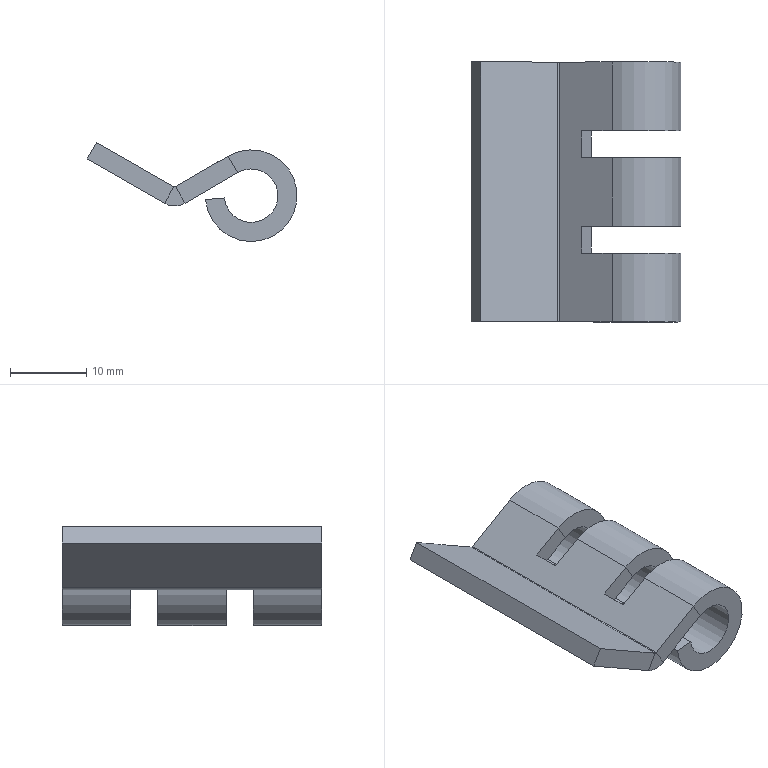Component | SolidWorks | FrontDoorFlangeWelding-2_CL201-1Hinge(ClawTypeAttachment)-1 | 1 solid | 34 faces | box 27.45 x 34 x 12.97 mm | volume 3368 mm3 | plane 26 | cylinder 8 | commonest cylinder face diameters 12 x3 7 x3 5.4 x1 0.4 x1
STEP:
#1=COLOUR_RGB('',0.7922,0.8196,0.9333);
#2=FILL_AREA_STYLE_COLOUR('',#1);
#3=FILL_AREA_STYLE('',(#2));
#4=SURFACE_STYLE_FILL_AREA(#3);
#5=SURFACE_SIDE_STYLE('',(#4));
#6=SURFACE_STYLE_USAGE(.BOTH.,#5);
#7=PRESENTATION_STYLE_ASSIGNMENT((#6));
#8=CARTESIAN_POINT('',(3.428,27.109,53.649));
#9=VERTEX_POINT('',#8);
#10=CARTESIAN_POINT('',(3.311,27.109,53.425));
#11=VERTEX_POINT('',#10);
#12=CARTESIAN_POINT('',(3.547,27.109,53.445));
#13=DIRECTION('',(0.,1.,0.));
#14=DIRECTION('',(-0.8677,0.,0.4971));
#15=AXIS2_PLACEMENT_3D('',#12,#13,#14);
#16=CIRCLE('',#15,0.2362);
#17=EDGE_CURVE('',#9,#11,#16,.T.);
#18=ORIENTED_EDGE('',*,*,#17,.T.);
#19=CARTESIAN_POINT('',(3.311,27.463,53.425));
#20=VERTEX_POINT('',#19);
#21=CARTESIAN_POINT('',(3.311,27.956,53.425));
#22=DIRECTION('',(-0.,-1.,-0.));
#23=VECTOR('',#22,39.37);
#24=LINE('',#21,#23);
#25=EDGE_CURVE('',#20,#11,#24,.T.);
#26=ORIENTED_EDGE('',*,*,#25,.F.);
#27=CARTESIAN_POINT('',(3.428,27.463,53.649));
#28=VERTEX_POINT('',#27);
#29=CARTESIAN_POINT('',(3.547,27.463,53.445));
#30=DIRECTION('',(-0.,-1.,-0.));
#31=DIRECTION('',(-0.8677,0.,0.4971));
#32=AXIS2_PLACEMENT_3D('',#29,#30,#31);
#33=CIRCLE('',#32,0.2362);
#34=EDGE_CURVE('',#20,#28,#33,.T.);
#35=ORIENTED_EDGE('',*,*,#34,.T.);
#36=CARTESIAN_POINT('',(3.428,27.956,53.649));
#37=DIRECTION('',(-0.,-1.,-0.));
#38=VECTOR('',#37,39.37);
#39=LINE('',#36,#38);
#40=EDGE_CURVE('',#28,#9,#39,.T.);
#41=ORIENTED_EDGE('',*,*,#40,.T.);
#42=EDGE_LOOP('',(#18,#26,#35,#41));
#43=FACE_OUTER_BOUND('',#42,.T.);
#44=CARTESIAN_POINT('',(3.547,27.956,53.445));
#45=DIRECTION('',(-0.,-1.,-0.));
#46=DIRECTION('',(-0.8677,0.,0.4971));
#47=AXIS2_PLACEMENT_3D('',#44,#45,#46);
#48=CYLINDRICAL_SURFACE('',#47,0.2362);
#49=ADVANCED_FACE('',(#43),#48,.T.);
#50=CARTESIAN_POINT('',(3.311,26.971,53.425));
#51=VERTEX_POINT('',#50);
#52=CARTESIAN_POINT('',(3.428,26.971,53.649));
#53=VERTEX_POINT('',#52);
#54=CARTESIAN_POINT('',(3.547,26.971,53.445));
#55=DIRECTION('',(-0.,-1.,-0.));
#56=DIRECTION('',(-0.8677,0.,0.4971));
#57=AXIS2_PLACEMENT_3D('',#54,#55,#56);
#58=CIRCLE('',#57,0.2362);
#59=EDGE_CURVE('',#51,#53,#58,.T.);
#60=ORIENTED_EDGE('',*,*,#59,.T.);
#61=CARTESIAN_POINT('',(3.428,26.617,53.649));
#62=VERTEX_POINT('',#61);
#63=CARTESIAN_POINT('',(3.428,27.956,53.649));
#64=DIRECTION('',(-0.,-1.,-0.));
#65=VECTOR('',#64,39.37);
#66=LINE('',#63,#65);
#67=EDGE_CURVE('',#53,#62,#66,.T.);
#68=ORIENTED_EDGE('',*,*,#67,.T.);
#69=CARTESIAN_POINT('',(3.311,26.617,53.425));
#70=VERTEX_POINT('',#69);
#71=CARTESIAN_POINT('',(3.547,26.617,53.445));
#72=DIRECTION('',(0.,1.,0.));
#73=DIRECTION('',(0.8677,0.,-0.4971));
#74=AXIS2_PLACEMENT_3D('',#71,#72,#73);
#75=CIRCLE('',#74,0.2362);
#76=EDGE_CURVE('',#62,#70,#75,.T.);
#77=ORIENTED_EDGE('',*,*,#76,.T.);
#78=CARTESIAN_POINT('',(3.311,27.956,53.425));
#79=DIRECTION('',(-0.,-1.,-0.));
#80=VECTOR('',#79,39.37);
#81=LINE('',#78,#80);
#82=EDGE_CURVE('',#51,#70,#81,.T.);
#83=ORIENTED_EDGE('',*,*,#82,.F.);
#84=EDGE_LOOP('',(#60,#68,#77,#83));
#85=FACE_OUTER_BOUND('',#84,.T.);
#86=CARTESIAN_POINT('',(3.547,27.956,53.445));
#87=DIRECTION('',(-0.,-1.,-0.));
#88=DIRECTION('',(-0.8677,0.,0.4971));
#89=AXIS2_PLACEMENT_3D('',#86,#87,#88);
#90=CYLINDRICAL_SURFACE('',#89,0.2362);
#91=ADVANCED_FACE('',(#85),#90,.T.);
#92=ORIENTED_EDGE('',*,*,#25,.T.);
#93=CARTESIAN_POINT('',(3.409,27.109,53.434));
#94=VERTEX_POINT('',#93);
#95=CARTESIAN_POINT('',(3.409,27.109,53.434));
#96=DIRECTION('',(-0.9965,0.,-0.08389));
#97=VECTOR('',#96,39.37);
#98=LINE('',#95,#97);
#99=EDGE_CURVE('',#94,#11,#98,.T.);
#100=ORIENTED_EDGE('',*,*,#99,.F.);
#101=CARTESIAN_POINT('',(3.409,27.463,53.434));
#102=VERTEX_POINT('',#101);
#103=CARTESIAN_POINT('',(3.409,27.956,53.434));
#104=DIRECTION('',(-0.,-1.,-0.));
#105=VECTOR('',#104,39.37);
#106=LINE('',#103,#105);
#107=EDGE_CURVE('',#102,#94,#106,.T.);
#108=ORIENTED_EDGE('',*,*,#107,.F.);
#109=CARTESIAN_POINT('',(3.409,27.463,53.434));
#110=DIRECTION('',(-0.9965,0.,-0.08389));
#111=VECTOR('',#110,39.37);
#112=LINE('',#109,#111);
#113=EDGE_CURVE('',#102,#20,#112,.T.);
#114=ORIENTED_EDGE('',*,*,#113,.T.);
#115=EDGE_LOOP('',(#92,#100,#108,#114));
#116=FACE_OUTER_BOUND('',#115,.T.);
#117=CARTESIAN_POINT('',(3.409,27.956,53.434));
#118=DIRECTION('',(-0.08389,-0.,0.9965));
#119=DIRECTION('',(0.9965,-0.,0.08389));
#120=AXIS2_PLACEMENT_3D('',#117,#118,#119);
#121=PLANE('',#120);
#122=ADVANCED_FACE('',(#116),#121,.T.);
#123=CARTESIAN_POINT('',(3.409,26.971,53.434));
#124=VERTEX_POINT('',#123);
#125=CARTESIAN_POINT('',(3.409,26.617,53.434));
#126=VERTEX_POINT('',#125);
#127=CARTESIAN_POINT('',(3.409,27.956,53.434));
#128=DIRECTION('',(-0.,-1.,-0.));
#129=VECTOR('',#128,39.37);
#130=LINE('',#127,#129);
#131=EDGE_CURVE('',#124,#126,#130,.T.);
#132=ORIENTED_EDGE('',*,*,#131,.F.);
#133=CARTESIAN_POINT('',(3.409,26.971,53.434));
#134=DIRECTION('',(-0.9965,0.,-0.08389));
#135=VECTOR('',#134,39.37);
#136=LINE('',#133,#135);
#137=EDGE_CURVE('',#124,#51,#136,.T.);
#138=ORIENTED_EDGE('',*,*,#137,.T.);
#139=ORIENTED_EDGE('',*,*,#82,.T.);
#140=CARTESIAN_POINT('',(3.409,26.617,53.434));
#141=DIRECTION('',(-0.9965,0.,-0.08389));
#142=VECTOR('',#141,39.37);
#143=LINE('',#140,#142);
#144=EDGE_CURVE('',#126,#70,#143,.T.);
#145=ORIENTED_EDGE('',*,*,#144,.F.);
#146=EDGE_LOOP('',(#132,#138,#139,#145));
#147=FACE_OUTER_BOUND('',#146,.T.);
#148=CARTESIAN_POINT('',(3.409,27.956,53.434));
#149=DIRECTION('',(-0.08389,-0.,0.9965));
#150=DIRECTION('',(0.9965,-0.,0.08389));
#151=AXIS2_PLACEMENT_3D('',#148,#149,#150);
#152=PLANE('',#151);
#153=ADVANCED_FACE('',(#147),#152,.T.);
#154=ORIENTED_EDGE('',*,*,#107,.T.);
#155=CARTESIAN_POINT('',(3.477,27.109,53.564));
#156=VERTEX_POINT('',#155);
#157=CARTESIAN_POINT('',(3.547,27.109,53.445));
#158=DIRECTION('',(0.,1.,0.));
#159=DIRECTION('',(0.8677,0.,-0.4971));
#160=AXIS2_PLACEMENT_3D('',#157,#158,#159);
#161=CIRCLE('',#160,0.1378);
#162=EDGE_CURVE('',#156,#94,#161,.T.);
#163=ORIENTED_EDGE('',*,*,#162,.F.);
#164=CARTESIAN_POINT('',(3.477,27.463,53.564));
#165=VERTEX_POINT('',#164);
#166=CARTESIAN_POINT('',(3.477,27.956,53.564));
#167=DIRECTION('',(-0.,-1.,-0.));
#168=VECTOR('',#167,39.37);
#169=LINE('',#166,#168);
#170=EDGE_CURVE('',#165,#156,#169,.T.);
#171=ORIENTED_EDGE('',*,*,#170,.F.);
#172=CARTESIAN_POINT('',(3.547,27.463,53.445));
#173=DIRECTION('',(-0.,-1.,-0.));
#174=DIRECTION('',(-0.8677,0.,0.4971));
#175=AXIS2_PLACEMENT_3D('',#172,#173,#174);
#176=CIRCLE('',#175,0.1378);
#177=EDGE_CURVE('',#102,#165,#176,.T.);
#178=ORIENTED_EDGE('',*,*,#177,.F.);
#179=EDGE_LOOP('',(#154,#163,#171,#178));
#180=FACE_OUTER_BOUND('',#179,.T.);
#181=CARTESIAN_POINT('',(3.547,27.956,53.445));
#182=DIRECTION('',(-0.,-1.,-0.));
#183=DIRECTION('',(-0.8677,0.,0.4971));
#184=AXIS2_PLACEMENT_3D('',#181,#182,#183);
#185=CYLINDRICAL_SURFACE('',#184,0.1378);
#186=ADVANCED_FACE('',(#180),#185,.F.);
#187=CARTESIAN_POINT('',(3.477,26.971,53.564));
#188=VERTEX_POINT('',#187);
#189=CARTESIAN_POINT('',(3.477,26.617,53.564));
#190=VERTEX_POINT('',#189);
#191=CARTESIAN_POINT('',(3.477,27.956,53.564));
#192=DIRECTION('',(-0.,-1.,-0.));
#193=VECTOR('',#192,39.37);
#194=LINE('',#191,#193);
#195=EDGE_CURVE('',#188,#190,#194,.T.);
#196=ORIENTED_EDGE('',*,*,#195,.F.);
#197=CARTESIAN_POINT('',(3.547,26.971,53.445));
#198=DIRECTION('',(0.,-1.,-0.));
#199=DIRECTION('',(-0.8677,0.,0.4971));
#200=AXIS2_PLACEMENT_3D('',#197,#198,#199);
#201=CIRCLE('',#200,0.1378);
#202=EDGE_CURVE('',#124,#188,#201,.T.);
#203=ORIENTED_EDGE('',*,*,#202,.F.);
#204=ORIENTED_EDGE('',*,*,#131,.T.);
#205=CARTESIAN_POINT('',(3.547,26.617,53.445));
#206=DIRECTION('',(0.,1.,0.));
#207=DIRECTION('',(0.8677,0.,-0.4971));
#208=AXIS2_PLACEMENT_3D('',#205,#206,#207);
#209=CIRCLE('',#208,0.1378);
#210=EDGE_CURVE('',#190,#126,#209,.T.);
#211=ORIENTED_EDGE('',*,*,#210,.F.);
#212=EDGE_LOOP('',(#196,#203,#204,#211));
#213=FACE_OUTER_BOUND('',#212,.T.);
#214=CARTESIAN_POINT('',(3.547,27.956,53.445));
#215=DIRECTION('',(-0.,-1.,-0.));
#216=DIRECTION('',(-0.8677,0.,0.4971));
#217=AXIS2_PLACEMENT_3D('',#214,#215,#216);
#218=CYLINDRICAL_SURFACE('',#217,0.1378);
#219=ADVANCED_FACE('',(#213),#218,.F.);
#220=ORIENTED_EDGE('',*,*,#170,.T.);
#221=CARTESIAN_POINT('',(3.32,27.109,53.473));
#222=VERTEX_POINT('',#221);
#223=CARTESIAN_POINT('',(3.153,27.109,53.376));
#224=DIRECTION('',(0.8644,-0.,0.5029));
#225=VECTOR('',#224,39.37);
#226=LINE('',#223,#225);
#227=EDGE_CURVE('',#222,#156,#226,.T.);
#228=ORIENTED_EDGE('',*,*,#227,.F.);
#229=CARTESIAN_POINT('',(3.32,26.971,53.473));
#230=VERTEX_POINT('',#229);
#231=CARTESIAN_POINT('',(3.32,27.956,53.473));
#232=DIRECTION('',(0.,1.,0.));
#233=VECTOR('',#232,39.37);
#234=LINE('',#231,#233);
#235=EDGE_CURVE('',#230,#222,#234,.T.);
#236=ORIENTED_EDGE('',*,*,#235,.F.);
#237=CARTESIAN_POINT('',(3.153,26.971,53.376));
#238=DIRECTION('',(-0.8644,0.,-0.5029));
#239=VECTOR('',#238,39.37);
#240=LINE('',#237,#239);
#241=EDGE_CURVE('',#188,#230,#240,.T.);
#242=ORIENTED_EDGE('',*,*,#241,.F.);
#243=ORIENTED_EDGE('',*,*,#195,.T.);
#244=CARTESIAN_POINT('',(3.206,26.617,53.406));
#245=VERTEX_POINT('',#244);
#246=CARTESIAN_POINT('',(3.153,26.617,53.376));
#247=DIRECTION('',(0.8644,-0.,0.5029));
#248=VECTOR('',#247,39.37);
#249=LINE('',#246,#248);
#250=EDGE_CURVE('',#245,#190,#249,.T.);
#251=ORIENTED_EDGE('',*,*,#250,.F.);
#252=CARTESIAN_POINT('',(3.206,27.956,53.406));
#253=VERTEX_POINT('',#252);
#254=CARTESIAN_POINT('',(3.206,27.956,53.406));
#255=DIRECTION('',(-0.,-1.,-0.));
#256=VECTOR('',#255,39.37);
#257=LINE('',#254,#256);
#258=EDGE_CURVE('',#253,#245,#257,.T.);
#259=ORIENTED_EDGE('',*,*,#258,.F.);
#260=CARTESIAN_POINT('',(3.477,27.956,53.564));
#261=VERTEX_POINT('',#260);
#262=CARTESIAN_POINT('',(3.153,27.956,53.376));
#263=DIRECTION('',(0.8644,-0.,0.5029));
#264=VECTOR('',#263,39.37);
#265=LINE('',#262,#264);
#266=EDGE_CURVE('',#253,#261,#265,.T.);
#267=ORIENTED_EDGE('',*,*,#266,.T.);
#268=CARTESIAN_POINT('',(3.477,27.601,53.564));
#269=VERTEX_POINT('',#268);
#270=CARTESIAN_POINT('',(3.477,27.956,53.564));
#271=DIRECTION('',(-0.,-1.,-0.));
#272=VECTOR('',#271,39.37);
#273=LINE('',#270,#272);
#274=EDGE_CURVE('',#261,#269,#273,.T.);
#275=ORIENTED_EDGE('',*,*,#274,.T.);
#276=CARTESIAN_POINT('',(3.32,27.601,53.473));
#277=VERTEX_POINT('',#276);
#278=CARTESIAN_POINT('',(3.153,27.601,53.376));
#279=DIRECTION('',(0.8644,-0.,0.5029));
#280=VECTOR('',#279,39.37);
#281=LINE('',#278,#280);
#282=EDGE_CURVE('',#277,#269,#281,.T.);
#283=ORIENTED_EDGE('',*,*,#282,.F.);
#284=CARTESIAN_POINT('',(3.32,27.463,53.473));
#285=VERTEX_POINT('',#284);
#286=CARTESIAN_POINT('',(3.32,27.956,53.473));
#287=DIRECTION('',(-0.,1.,0.));
#288=VECTOR('',#287,39.37);
#289=LINE('',#286,#288);
#290=EDGE_CURVE('',#285,#277,#289,.T.);
#291=ORIENTED_EDGE('',*,*,#290,.F.);
#292=CARTESIAN_POINT('',(3.153,27.463,53.376));
#293=DIRECTION('',(-0.8644,0.,-0.5029));
#294=VECTOR('',#293,39.37);
#295=LINE('',#292,#294);
#296=EDGE_CURVE('',#165,#285,#295,.T.);
#297=ORIENTED_EDGE('',*,*,#296,.F.);
#298=EDGE_LOOP('',(#220,#228,#236,#242,#243,#251,#259,#267,#275,#283,#291,#297));
#299=FACE_OUTER_BOUND('',#298,.T.);
#300=CARTESIAN_POINT('',(3.153,27.956,53.376));
#301=DIRECTION('',(0.5029,0.,-0.8644));
#302=DIRECTION('',(-0.8644,0.,-0.5029));
#303=AXIS2_PLACEMENT_3D('',#300,#301,#302);
#304=PLANE('',#303);
#305=ADVANCED_FACE('',(#299),#304,.T.);
#306=CARTESIAN_POINT('',(3.271,27.109,53.558));
#307=VERTEX_POINT('',#306);
#308=CARTESIAN_POINT('',(3.104,27.109,53.461));
#309=DIRECTION('',(0.8644,-0.,0.5029));
#310=VECTOR('',#309,39.37);
#311=LINE('',#308,#310);
#312=EDGE_CURVE('',#307,#9,#311,.T.);
#313=ORIENTED_EDGE('',*,*,#312,.T.);
#314=ORIENTED_EDGE('',*,*,#40,.F.);
#315=CARTESIAN_POINT('',(3.271,27.463,53.558));
#316=VERTEX_POINT('',#315);
#317=CARTESIAN_POINT('',(3.104,27.463,53.461));
#318=DIRECTION('',(-0.8644,0.,-0.5029));
#319=VECTOR('',#318,39.37);
#320=LINE('',#317,#319);
#321=EDGE_CURVE('',#28,#316,#320,.T.);
#322=ORIENTED_EDGE('',*,*,#321,.T.);
#323=CARTESIAN_POINT('',(3.271,27.601,53.558));
#324=VERTEX_POINT('',#323);
#325=CARTESIAN_POINT('',(3.271,27.956,53.558));
#326=DIRECTION('',(0.,1.,0.));
#327=VECTOR('',#326,39.37);
#328=LINE('',#325,#327);
#329=EDGE_CURVE('',#316,#324,#328,.T.);
#330=ORIENTED_EDGE('',*,*,#329,.T.);
#331=CARTESIAN_POINT('',(3.428,27.601,53.649));
#332=VERTEX_POINT('',#331);
#333=CARTESIAN_POINT('',(3.104,27.601,53.461));
#334=DIRECTION('',(0.8644,-0.,0.5029));
#335=VECTOR('',#334,39.37);
#336=LINE('',#333,#335);
#337=EDGE_CURVE('',#324,#332,#336,.T.);
#338=ORIENTED_EDGE('',*,*,#337,.T.);
#339=CARTESIAN_POINT('',(3.428,27.956,53.649));
#340=VERTEX_POINT('',#339);
#341=CARTESIAN_POINT('',(3.428,27.956,53.649));
#342=DIRECTION('',(-0.,-1.,-0.));
#343=VECTOR('',#342,39.37);
#344=LINE('',#341,#343);
#345=EDGE_CURVE('',#340,#332,#344,.T.);
#346=ORIENTED_EDGE('',*,*,#345,.F.);
#347=CARTESIAN_POINT('',(3.157,27.956,53.492));
#348=VERTEX_POINT('',#347);
#349=CARTESIAN_POINT('',(3.104,27.956,53.461));
#350=DIRECTION('',(0.8644,-0.,0.5029));
#351=VECTOR('',#350,39.37);
#352=LINE('',#349,#351);
#353=EDGE_CURVE('',#348,#340,#352,.T.);
#354=ORIENTED_EDGE('',*,*,#353,.F.);
#355=CARTESIAN_POINT('',(3.157,26.617,53.492));
#356=VERTEX_POINT('',#355);
#357=CARTESIAN_POINT('',(3.157,27.956,53.492));
#358=DIRECTION('',(-0.,-1.,-0.));
#359=VECTOR('',#358,39.37);
#360=LINE('',#357,#359);
#361=EDGE_CURVE('',#348,#356,#360,.T.);
#362=ORIENTED_EDGE('',*,*,#361,.T.);
#363=CARTESIAN_POINT('',(3.104,26.617,53.461));
#364=DIRECTION('',(0.8644,-0.,0.5029));
#365=VECTOR('',#364,39.37);
#366=LINE('',#363,#365);
#367=EDGE_CURVE('',#356,#62,#366,.T.);
#368=ORIENTED_EDGE('',*,*,#367,.T.);
#369=ORIENTED_EDGE('',*,*,#67,.F.);
#370=CARTESIAN_POINT('',(3.271,26.971,53.558));
#371=VERTEX_POINT('',#370);
#372=CARTESIAN_POINT('',(3.104,26.971,53.461));
#373=DIRECTION('',(-0.8644,0.,-0.5029));
#374=VECTOR('',#373,39.37);
#375=LINE('',#372,#374);
#376=EDGE_CURVE('',#53,#371,#375,.T.);
#377=ORIENTED_EDGE('',*,*,#376,.T.);
#378=CARTESIAN_POINT('',(3.271,27.956,53.558));
#379=DIRECTION('',(0.,1.,0.));
#380=VECTOR('',#379,39.37);
#381=LINE('',#378,#380);
#382=EDGE_CURVE('',#371,#307,#381,.T.);
#383=ORIENTED_EDGE('',*,*,#382,.T.);
#384=EDGE_LOOP('',(#313,#314,#322,#330,#338,#346,#354,#362,#368,#369,#377,#383));
#385=FACE_OUTER_BOUND('',#384,.T.);
#386=CARTESIAN_POINT('',(3.104,27.956,53.461));
#387=DIRECTION('',(0.5029,0.,-0.8644));
#388=DIRECTION('',(-0.8644,0.,-0.5029));
#389=AXIS2_PLACEMENT_3D('',#386,#387,#388);
#390=PLANE('',#389);
#391=ADVANCED_FACE('',(#385),#390,.F.);
#392=CARTESIAN_POINT('',(3.311,27.601,53.425));
#393=VERTEX_POINT('',#392);
#394=CARTESIAN_POINT('',(3.547,27.601,53.445));
#395=DIRECTION('',(0.,1.,0.));
#396=DIRECTION('',(-0.8677,0.,0.4971));
#397=AXIS2_PLACEMENT_3D('',#394,#395,#396);
#398=CIRCLE('',#397,0.2362);
#399=EDGE_CURVE('',#332,#393,#398,.T.);
#400=ORIENTED_EDGE('',*,*,#399,.T.);
#401=CARTESIAN_POINT('',(3.311,27.956,53.425));
#402=VERTEX_POINT('',#401);
#403=CARTESIAN_POINT('',(3.311,27.956,53.425));
#404=DIRECTION('',(-0.,-1.,-0.));
#405=VECTOR('',#404,39.37);
#406=LINE('',#403,#405);
#407=EDGE_CURVE('',#402,#393,#406,.T.);
#408=ORIENTED_EDGE('',*,*,#407,.F.);
#409=CARTESIAN_POINT('',(3.547,27.956,53.445));
#410=DIRECTION('',(0.,1.,0.));
#411=DIRECTION('',(0.8677,0.,-0.4971));
#412=AXIS2_PLACEMENT_3D('',#409,#410,#411);
#413=CIRCLE('',#412,0.2362);
#414=EDGE_CURVE('',#340,#402,#413,.T.);
#415=ORIENTED_EDGE('',*,*,#414,.F.);
#416=ORIENTED_EDGE('',*,*,#345,.T.);
#417=EDGE_LOOP('',(#400,#408,#415,#416));
#418=FACE_OUTER_BOUND('',#417,.T.);
#419=CARTESIAN_POINT('',(3.547,27.956,53.445));
#420=DIRECTION('',(-0.,-1.,-0.));
#421=DIRECTION('',(-0.8677,0.,0.4971));
#422=AXIS2_PLACEMENT_3D('',#419,#420,#421);
#423=CYLINDRICAL_SURFACE('',#422,0.2362);
#424=ADVANCED_FACE('',(#418),#423,.T.);
#425=ORIENTED_EDGE('',*,*,#407,.T.);
#426=CARTESIAN_POINT('',(3.409,27.601,53.434));
#427=VERTEX_POINT('',#426);
#428=CARTESIAN_POINT('',(3.409,27.601,53.434));
#429=DIRECTION('',(-0.9965,0.,-0.08389));
#430=VECTOR('',#429,39.37);
#431=LINE('',#428,#430);
#432=EDGE_CURVE('',#427,#393,#431,.T.);
#433=ORIENTED_EDGE('',*,*,#432,.F.);
#434=CARTESIAN_POINT('',(3.409,27.956,53.434));
#435=VERTEX_POINT('',#434);
#436=CARTESIAN_POINT('',(3.409,27.956,53.434));
#437=DIRECTION('',(-0.,-1.,-0.));
#438=VECTOR('',#437,39.37);
#439=LINE('',#436,#438);
#440=EDGE_CURVE('',#435,#427,#439,.T.);
#441=ORIENTED_EDGE('',*,*,#440,.F.);
#442=CARTESIAN_POINT('',(3.409,27.956,53.434));
#443=DIRECTION('',(-0.9965,0.,-0.08389));
#444=VECTOR('',#443,39.37);
#445=LINE('',#442,#444);
#446=EDGE_CURVE('',#435,#402,#445,.T.);
#447=ORIENTED_EDGE('',*,*,#446,.T.);
#448=EDGE_LOOP('',(#425,#433,#441,#447));
#449=FACE_OUTER_BOUND('',#448,.T.);
#450=CARTESIAN_POINT('',(3.409,27.956,53.434));
#451=DIRECTION('',(-0.08389,-0.,0.9965));
#452=DIRECTION('',(0.9965,-0.,0.08389));
#453=AXIS2_PLACEMENT_3D('',#450,#451,#452);
#454=PLANE('',#453);
#455=ADVANCED_FACE('',(#449),#454,.T.);
#456=ORIENTED_EDGE('',*,*,#440,.T.);
#457=CARTESIAN_POINT('',(3.547,27.601,53.445));
#458=DIRECTION('',(0.,1.,0.));
#459=DIRECTION('',(0.8677,0.,-0.4971));
#460=AXIS2_PLACEMENT_3D('',#457,#458,#459);
#461=CIRCLE('',#460,0.1378);
#462=EDGE_CURVE('',#269,#427,#461,.T.);
#463=ORIENTED_EDGE('',*,*,#462,.F.);
#464=ORIENTED_EDGE('',*,*,#274,.F.);
#465=CARTESIAN_POINT('',(3.547,27.956,53.445));
#466=DIRECTION('',(0.,1.,0.));
#467=DIRECTION('',(0.8677,0.,-0.4971));
#468=AXIS2_PLACEMENT_3D('',#465,#466,#467);
#469=CIRCLE('',#468,0.1378);
#470=EDGE_CURVE('',#261,#435,#469,.T.);
#471=ORIENTED_EDGE('',*,*,#470,.T.);
#472=EDGE_LOOP('',(#456,#463,#464,#471));
#473=FACE_OUTER_BOUND('',#472,.T.);
#474=CARTESIAN_POINT('',(3.547,27.956,53.445));
#475=DIRECTION('',(-0.,-1.,-0.));
#476=DIRECTION('',(-0.8677,0.,0.4971));
#477=AXIS2_PLACEMENT_3D('',#474,#475,#476);
#478=CYLINDRICAL_SURFACE('',#477,0.1378);
#479=ADVANCED_FACE('',(#473),#478,.F.);
#480=CARTESIAN_POINT('',(3.428,27.956,53.649));
#481=DIRECTION('',(0.5029,0.,-0.8644));
#482=VECTOR('',#481,39.37);
#483=LINE('',#480,#482);
#484=EDGE_CURVE('',#340,#261,#483,.T.);
#485=ORIENTED_EDGE('',*,*,#484,.F.);
#486=ORIENTED_EDGE('',*,*,#414,.T.);
#487=ORIENTED_EDGE('',*,*,#446,.F.);
#488=ORIENTED_EDGE('',*,*,#470,.F.);
#489=EDGE_LOOP('',(#485,#486,#487,#488));
#490=FACE_OUTER_BOUND('',#489,.T.);
#491=CARTESIAN_POINT('',(3.428,27.956,53.649));
#492=DIRECTION('',(0.,1.,0.));
#493=DIRECTION('',(0.8677,0.,-0.4971));
#494=AXIS2_PLACEMENT_3D('',#491,#492,#493);
#495=PLANE('',#494);
#496=ADVANCED_FACE('',(#490),#495,.T.);
#497=CARTESIAN_POINT('',(3.477,26.617,53.564));
#498=DIRECTION('',(-0.5029,-0.,0.8644));
#499=VECTOR('',#498,39.37);
#500=LINE('',#497,#499);
#501=EDGE_CURVE('',#190,#62,#500,.T.);
#502=ORIENTED_EDGE('',*,*,#501,.F.);
#503=ORIENTED_EDGE('',*,*,#210,.T.);
#504=ORIENTED_EDGE('',*,*,#144,.T.);
#505=ORIENTED_EDGE('',*,*,#76,.F.);
#506=EDGE_LOOP('',(#502,#503,#504,#505));
#507=FACE_OUTER_BOUND('',#506,.T.);
#508=CARTESIAN_POINT('',(3.477,26.617,53.564));
#509=DIRECTION('',(-0.,-1.,-0.));
#510=DIRECTION('',(-0.8677,-0.,0.4971));
#511=AXIS2_PLACEMENT_3D('',#508,#509,#510);
#512=PLANE('',#511);
#513=ADVANCED_FACE('',(#507),#512,.T.);
#514=CARTESIAN_POINT('',(3.206,27.956,53.406));
#515=DIRECTION('',(-0.5029,-0.,0.8644));
#516=VECTOR('',#515,39.37);
#517=LINE('',#514,#516);
#518=EDGE_CURVE('',#253,#348,#517,.T.);
#519=ORIENTED_EDGE('',*,*,#518,.F.);
#520=CARTESIAN_POINT('',(3.1,27.956,53.406));
#521=VERTEX_POINT('',#520);
#522=CARTESIAN_POINT('',(3.153,27.956,53.498));
#523=DIRECTION('',(-0.,-1.,-0.));
#524=DIRECTION('',(0.8677,0.,-0.4971));
#525=AXIS2_PLACEMENT_3D('',#522,#523,#524);
#526=CIRCLE('',#525,0.1063);
#527=EDGE_CURVE('',#521,#253,#526,.T.);
#528=ORIENTED_EDGE('',*,*,#527,.F.);
#529=CARTESIAN_POINT('',(3.149,27.956,53.492));
#530=VERTEX_POINT('',#529);
#531=CARTESIAN_POINT('',(3.149,27.956,53.492));
#532=DIRECTION('',(-0.4971,0.,-0.8677));
#533=VECTOR('',#532,39.37);
#534=LINE('',#531,#533);
#535=EDGE_CURVE('',#530,#521,#534,.T.);
#536=ORIENTED_EDGE('',*,*,#535,.F.);
#537=CARTESIAN_POINT('',(3.153,27.956,53.498));
#538=DIRECTION('',(-0.,-1.,-0.));
#539=DIRECTION('',(0.8677,0.,-0.4971));
#540=AXIS2_PLACEMENT_3D('',#537,#538,#539);
#541=CIRCLE('',#540,0.007874);
#542=EDGE_CURVE('',#530,#348,#541,.T.);
#543=ORIENTED_EDGE('',*,*,#542,.T.);
#544=EDGE_LOOP('',(#519,#528,#536,#543));
#545=FACE_OUTER_BOUND('',#544,.T.);
#546=CARTESIAN_POINT('',(3.206,27.956,53.406));
#547=DIRECTION('',(0.,1.,0.));
#548=DIRECTION('',(0.8677,0.,-0.4971));
#549=AXIS2_PLACEMENT_3D('',#546,#547,#548);
#550=PLANE('',#549);
#551=ADVANCED_FACE('',(#545),#550,.T.);
#552=ORIENTED_EDGE('',*,*,#266,.F.);
#553=ORIENTED_EDGE('',*,*,#518,.T.);
#554=ORIENTED_EDGE('',*,*,#353,.T.);
#555=ORIENTED_EDGE('',*,*,#484,.T.);
#556=EDGE_LOOP('',(#552,#553,#554,#555));
#557=FACE_OUTER_BOUND('',#556,.T.);
#558=CARTESIAN_POINT('',(3.149,27.956,53.492));
#559=DIRECTION('',(0.,1.,0.));
#560=DIRECTION('',(0.8677,0.,-0.4971));
#561=AXIS2_PLACEMENT_3D('',#558,#559,#560);
#562=PLANE('',#561);
#563=ADVANCED_FACE('',(#557),#562,.T.);
#564=CARTESIAN_POINT('',(3.1,26.617,53.406));
#565=VERTEX_POINT('',#564);
#566=CARTESIAN_POINT('',(3.149,26.617,53.492));
#567=VERTEX_POINT('',#566);
#568=CARTESIAN_POINT('',(3.1,26.617,53.406));
#569=DIRECTION('',(0.4971,-0.,0.8677));
#570=VECTOR('',#569,39.37);
#571=LINE('',#568,#570);
#572=EDGE_CURVE('',#565,#567,#571,.T.);
#573=ORIENTED_EDGE('',*,*,#572,.F.);
#574=CARTESIAN_POINT('',(3.153,26.617,53.498));
#575=DIRECTION('',(-0.,-1.,-0.));
#576=DIRECTION('',(0.8677,0.,-0.4971));
#577=AXIS2_PLACEMENT_3D('',#574,#575,#576);
#578=CIRCLE('',#577,0.1063);
#579=EDGE_CURVE('',#565,#245,#578,.T.);
#580=ORIENTED_EDGE('',*,*,#579,.T.);
#581=CARTESIAN_POINT('',(3.157,26.617,53.492));
#582=DIRECTION('',(0.5029,0.,-0.8644));
#583=VECTOR('',#582,39.37);
#584=LINE('',#581,#583);
#585=EDGE_CURVE('',#356,#245,#584,.T.);
#586=ORIENTED_EDGE('',*,*,#585,.F.);
#587=CARTESIAN_POINT('',(3.153,26.617,53.498));
#588=DIRECTION('',(-0.,-1.,-0.));
#589=DIRECTION('',(0.8677,0.,-0.4971));
#590=AXIS2_PLACEMENT_3D('',#587,#588,#589);
#591=CIRCLE('',#590,0.007874);
#592=EDGE_CURVE('',#567,#356,#591,.T.);
#593=ORIENTED_EDGE('',*,*,#592,.F.);
#594=EDGE_LOOP('',(#573,#580,#586,#593));
#595=FACE_OUTER_BOUND('',#594,.T.);
#596=CARTESIAN_POINT('',(3.1,26.617,53.406));
#597=DIRECTION('',(-0.,-1.,-0.));
#598=DIRECTION('',(-0.8677,-0.,0.4971));
#599=AXIS2_PLACEMENT_3D('',#596,#597,#598);
#600=PLANE('',#599);
#601=ADVANCED_FACE('',(#595),#600,.T.);
#602=CARTESIAN_POINT('',(2.702,26.617,53.634));
#603=VERTEX_POINT('',#602);
#604=CARTESIAN_POINT('',(2.702,26.617,53.634));
#605=DIRECTION('',(0.8677,0.,-0.4971));
#606=VECTOR('',#605,39.37);
#607=LINE('',#604,#606);
#608=EDGE_CURVE('',#603,#565,#607,.T.);
#609=ORIENTED_EDGE('',*,*,#608,.T.);
#610=ORIENTED_EDGE('',*,*,#572,.T.);
#611=CARTESIAN_POINT('',(2.751,26.617,53.719));
#612=VERTEX_POINT('',#611);
#613=CARTESIAN_POINT('',(2.751,26.617,53.719));
#614=DIRECTION('',(0.8677,0.,-0.4971));
#615=VECTOR('',#614,39.37);
#616=LINE('',#613,#615);
#617=EDGE_CURVE('',#612,#567,#616,.T.);
#618=ORIENTED_EDGE('',*,*,#617,.F.);
#619=CARTESIAN_POINT('',(2.751,26.617,53.719));
#620=DIRECTION('',(-0.4971,0.,-0.8677));
#621=VECTOR('',#620,39.37);
#622=LINE('',#619,#621);
#623=EDGE_CURVE('',#612,#603,#622,.T.);
#624=ORIENTED_EDGE('',*,*,#623,.T.);
#625=EDGE_LOOP('',(#609,#610,#618,#624));
#626=FACE_OUTER_BOUND('',#625,.T.);
#627=CARTESIAN_POINT('',(3.157,26.617,53.492));
#628=DIRECTION('',(-0.,-1.,-0.));
#629=DIRECTION('',(-0.8677,-0.,0.4971));
#630=AXIS2_PLACEMENT_3D('',#627,#628,#629);
#631=PLANE('',#630);
#632=ADVANCED_FACE('',(#626),#631,.T.);
#633=ORIENTED_EDGE('',*,*,#579,.F.);
#634=CARTESIAN_POINT('',(3.1,27.956,53.406));
#635=DIRECTION('',(-0.,-1.,-0.));
#636=VECTOR('',#635,39.37);
#637=LINE('',#634,#636);
#638=EDGE_CURVE('',#521,#565,#637,.T.);
#639=ORIENTED_EDGE('',*,*,#638,.F.);
#640=ORIENTED_EDGE('',*,*,#527,.T.);
#641=ORIENTED_EDGE('',*,*,#258,.T.);
#642=EDGE_LOOP('',(#633,#639,#640,#641));
#643=FACE_OUTER_BOUND('',#642,.T.);
#644=CARTESIAN_POINT('',(3.153,27.956,53.498));
#645=DIRECTION('',(-0.,-1.,-0.));
#646=DIRECTION('',(-0.8677,0.,0.4971));
#647=AXIS2_PLACEMENT_3D('',#644,#645,#646);
#648=CYLINDRICAL_SURFACE('',#647,0.1063);
#649=ADVANCED_FACE('',(#643),#648,.T.);
#650=ORIENTED_EDGE('',*,*,#608,.F.);
#651=CARTESIAN_POINT('',(2.702,27.956,53.634));
#652=VERTEX_POINT('',#651);
#653=CARTESIAN_POINT('',(2.702,27.956,53.634));
#654=DIRECTION('',(-0.,-1.,-0.));
#655=VECTOR('',#654,39.37);
#656=LINE('',#653,#655);
#657=EDGE_CURVE('',#652,#603,#656,.T.);
#658=ORIENTED_EDGE('',*,*,#657,.F.);
#659=CARTESIAN_POINT('',(2.702,27.956,53.634));
#660=DIRECTION('',(0.8677,0.,-0.4971));
#661=VECTOR('',#660,39.37);
#662=LINE('',#659,#661);
#663=EDGE_CURVE('',#652,#521,#662,.T.);
#664=ORIENTED_EDGE('',*,*,#663,.T.);
#665=ORIENTED_EDGE('',*,*,#638,.T.);
#666=EDGE_LOOP('',(#650,#658,#664,#665));
#667=FACE_OUTER_BOUND('',#666,.T.);
#668=CARTESIAN_POINT('',(2.702,27.956,53.634));
#669=DIRECTION('',(-0.4971,0.,-0.8677));
#670=DIRECTION('',(0.,1.,0.));
#671=AXIS2_PLACEMENT_3D('',#668,#669,#670);
#672=PLANE('',#671);
#673=ADVANCED_FACE('',(#667),#672,.T.);
#674=ORIENTED_EDGE('',*,*,#623,.F.);
#675=CARTESIAN_POINT('',(2.751,27.956,53.719));
#676=VERTEX_POINT('',#675);
#677=CARTESIAN_POINT('',(2.751,27.956,53.719));
#678=DIRECTION('',(-0.,-1.,-0.));
#679=VECTOR('',#678,39.37);
#680=LINE('',#677,#679);
#681=EDGE_CURVE('',#676,#612,#680,.T.);
#682=ORIENTED_EDGE('',*,*,#681,.F.);
#683=CARTESIAN_POINT('',(2.751,27.956,53.719));
#684=DIRECTION('',(-0.4971,0.,-0.8677));
#685=VECTOR('',#684,39.37);
#686=LINE('',#683,#685);
#687=EDGE_CURVE('',#676,#652,#686,.T.);
#688=ORIENTED_EDGE('',*,*,#687,.T.);
#689=ORIENTED_EDGE('',*,*,#657,.T.);
#690=EDGE_LOOP('',(#674,#682,#688,#689));
#691=FACE_OUTER_BOUND('',#690,.T.);
#692=CARTESIAN_POINT('',(2.751,27.956,53.719));
#693=DIRECTION('',(-0.8677,-0.,0.4971));
#694=DIRECTION('',(0.,1.,0.));
#695=AXIS2_PLACEMENT_3D('',#692,#693,#694);
#696=PLANE('',#695);
#697=ADVANCED_FACE('',(#691),#696,.T.);
#698=ORIENTED_EDGE('',*,*,#617,.T.);
#699=CARTESIAN_POINT('',(3.149,27.956,53.492));
#700=DIRECTION('',(-0.,-1.,-0.));
#701=VECTOR('',#700,39.37);
#702=LINE('',#699,#701);
#703=EDGE_CURVE('',#530,#567,#702,.T.);
#704=ORIENTED_EDGE('',*,*,#703,.F.);
#705=CARTESIAN_POINT('',(2.751,27.956,53.719));
#706=DIRECTION('',(0.8677,0.,-0.4971));
#707=VECTOR('',#706,39.37);
#708=LINE('',#705,#707);
#709=EDGE_CURVE('',#676,#530,#708,.T.);
#710=ORIENTED_EDGE('',*,*,#709,.F.);
#711=ORIENTED_EDGE('',*,*,#681,.T.);
#712=EDGE_LOOP('',(#698,#704,#710,#711));
#713=FACE_OUTER_BOUND('',#712,.T.);
#714=CARTESIAN_POINT('',(2.751,27.956,53.719));
#715=DIRECTION('',(-0.4971,0.,-0.8677));
#716=DIRECTION('',(0.,1.,0.));
#717=AXIS2_PLACEMENT_3D('',#714,#715,#716);
#718=PLANE('',#717);
#719=ADVANCED_FACE('',(#713),#718,.F.);
#720=ORIENTED_EDGE('',*,*,#592,.T.);
#721=ORIENTED_EDGE('',*,*,#361,.F.);
#722=ORIENTED_EDGE('',*,*,#542,.F.);
#723=ORIENTED_EDGE('',*,*,#703,.T.);
#724=EDGE_LOOP('',(#720,#721,#722,#723));
#725=FACE_OUTER_BOUND('',#724,.T.);
#726=CARTESIAN_POINT('',(3.153,27.956,53.498));
#727=DIRECTION('',(-0.,-1.,-0.));
#728=DIRECTION('',(-0.8677,0.,0.4971));
#729=AXIS2_PLACEMENT_3D('',#726,#727,#728);
#730=CYLINDRICAL_SURFACE('',#729,0.007874);
#731=ADVANCED_FACE('',(#725),#730,.F.);
#732=ORIENTED_EDGE('',*,*,#709,.T.);
#733=ORIENTED_EDGE('',*,*,#535,.T.);
#734=ORIENTED_EDGE('',*,*,#663,.F.);
#735=ORIENTED_EDGE('',*,*,#687,.F.);
#736=EDGE_LOOP('',(#732,#733,#734,#735));
#737=FACE_OUTER_BOUND('',#736,.T.);
#738=CARTESIAN_POINT('',(3.547,27.956,53.445));
#739=DIRECTION('',(0.,1.,0.));
#740=DIRECTION('',(0.8677,0.,-0.4971));
#741=AXIS2_PLACEMENT_3D('',#738,#739,#740);
#742=PLANE('',#741);
#743=ADVANCED_FACE('',(#737),#742,.T.);
#744=ORIENTED_EDGE('',*,*,#250,.T.);
#745=ORIENTED_EDGE('',*,*,#501,.T.);
#746=ORIENTED_EDGE('',*,*,#367,.F.);
#747=ORIENTED_EDGE('',*,*,#585,.T.);
#748=EDGE_LOOP('',(#744,#745,#746,#747));
#749=FACE_OUTER_BOUND('',#748,.T.);
#750=CARTESIAN_POINT('',(3.547,26.617,53.445));
#751=DIRECTION('',(0.,1.,0.));
#752=DIRECTION('',(0.8677,0.,-0.4971));
#753=AXIS2_PLACEMENT_3D('',#750,#751,#752);
#754=PLANE('',#753);
#755=ADVANCED_FACE('',(#749),#754,.F.);
#756=ORIENTED_EDGE('',*,*,#321,.F.);
#757=CARTESIAN_POINT('',(3.428,27.463,53.649));
#758=DIRECTION('',(0.5029,0.,-0.8644));
#759=VECTOR('',#758,39.37);
#760=LINE('',#757,#759);
#761=EDGE_CURVE('',#28,#165,#760,.T.);
#762=ORIENTED_EDGE('',*,*,#761,.T.);
#763=ORIENTED_EDGE('',*,*,#296,.T.);
#764=CARTESIAN_POINT('',(3.32,27.463,53.473));
#765=DIRECTION('',(-0.5029,-0.,0.8644));
#766=VECTOR('',#765,39.37);
#767=LINE('',#764,#766);
#768=EDGE_CURVE('',#285,#316,#767,.T.);
#769=ORIENTED_EDGE('',*,*,#768,.T.);
#770=EDGE_LOOP('',(#756,#762,#763,#769));
#771=FACE_OUTER_BOUND('',#770,.T.);
#772=CARTESIAN_POINT('',(3.104,27.463,53.461));
#773=DIRECTION('',(-0.,-1.,-0.));
#774=DIRECTION('',(-0.8644,0.,-0.5029));
#775=AXIS2_PLACEMENT_3D('',#772,#773,#774);
#776=PLANE('',#775);
#777=ADVANCED_FACE('',(#771),#776,.F.);
#778=CARTESIAN_POINT('',(3.428,27.601,53.649));
#779=DIRECTION('',(0.5029,0.,-0.8644));
#780=VECTOR('',#779,39.37);
#781=LINE('',#778,#780);
#782=EDGE_CURVE('',#332,#269,#781,.T.);
#783=ORIENTED_EDGE('',*,*,#782,.F.);
#784=ORIENTED_EDGE('',*,*,#337,.F.);
#785=CARTESIAN_POINT('',(3.32,27.601,53.473));
#786=DIRECTION('',(-0.5029,-0.,0.8644));
#787=VECTOR('',#786,39.37);
#788=LINE('',#785,#787);
#789=EDGE_CURVE('',#277,#324,#788,.T.);
#790=ORIENTED_EDGE('',*,*,#789,.F.);
#791=ORIENTED_EDGE('',*,*,#282,.T.);
#792=EDGE_LOOP('',(#783,#784,#790,#791));
#793=FACE_OUTER_BOUND('',#792,.T.);
#794=CARTESIAN_POINT('',(3.104,27.601,53.461));
#795=DIRECTION('',(0.,1.,0.));
#796=DIRECTION('',(0.8644,-0.,0.5029));
#797=AXIS2_PLACEMENT_3D('',#794,#795,#796);
#798=PLANE('',#797);
#799=ADVANCED_FACE('',(#793),#798,.F.);
#800=ORIENTED_EDGE('',*,*,#768,.F.);
#801=ORIENTED_EDGE('',*,*,#290,.T.);
#802=ORIENTED_EDGE('',*,*,#789,.T.);
#803=ORIENTED_EDGE('',*,*,#329,.F.);
#804=EDGE_LOOP('',(#800,#801,#802,#803));
#805=FACE_OUTER_BOUND('',#804,.T.);
#806=CARTESIAN_POINT('',(3.32,27.956,53.473));
#807=DIRECTION('',(-0.8644,0.,-0.5029));
#808=DIRECTION('',(-0.,1.,0.));
#809=AXIS2_PLACEMENT_3D('',#806,#807,#808);
#810=PLANE('',#809);
#811=ADVANCED_FACE('',(#805),#810,.F.);
#812=ORIENTED_EDGE('',*,*,#113,.F.);
#813=ORIENTED_EDGE('',*,*,#177,.T.);
#814=ORIENTED_EDGE('',*,*,#761,.F.);
#815=ORIENTED_EDGE('',*,*,#34,.F.);
#816=EDGE_LOOP('',(#812,#813,#814,#815));
#817=FACE_OUTER_BOUND('',#816,.T.);
#818=CARTESIAN_POINT('',(3.547,27.463,53.445));
#819=DIRECTION('',(0.,1.,0.));
#820=DIRECTION('',(0.8677,0.,-0.4971));
#821=AXIS2_PLACEMENT_3D('',#818,#819,#820);
#822=PLANE('',#821);
#823=ADVANCED_FACE('',(#817),#822,.T.);
#824=ORIENTED_EDGE('',*,*,#462,.T.);
#825=ORIENTED_EDGE('',*,*,#432,.T.);
#826=ORIENTED_EDGE('',*,*,#399,.F.);
#827=ORIENTED_EDGE('',*,*,#782,.T.);
#828=EDGE_LOOP('',(#824,#825,#826,#827));
#829=FACE_OUTER_BOUND('',#828,.T.);
#830=CARTESIAN_POINT('',(3.547,27.601,53.445));
#831=DIRECTION('',(-0.,-1.,-0.));
#832=DIRECTION('',(-0.8677,-0.,0.4971));
#833=AXIS2_PLACEMENT_3D('',#830,#831,#832);
#834=PLANE('',#833);
#835=ADVANCED_FACE('',(#829),#834,.T.);
#836=CARTESIAN_POINT('',(3.428,27.109,53.649));
#837=DIRECTION('',(0.5029,0.,-0.8644));
#838=VECTOR('',#837,39.37);
#839=LINE('',#836,#838);
#840=EDGE_CURVE('',#9,#156,#839,.T.);
#841=ORIENTED_EDGE('',*,*,#840,.F.);
#842=ORIENTED_EDGE('',*,*,#312,.F.);
#843=CARTESIAN_POINT('',(3.32,27.109,53.473));
#844=DIRECTION('',(-0.5029,-0.,0.8644));
#845=VECTOR('',#844,39.37);
#846=LINE('',#843,#845);
#847=EDGE_CURVE('',#222,#307,#846,.T.);
#848=ORIENTED_EDGE('',*,*,#847,.F.);
#849=ORIENTED_EDGE('',*,*,#227,.T.);
#850=EDGE_LOOP('',(#841,#842,#848,#849));
#851=FACE_OUTER_BOUND('',#850,.T.);
#852=CARTESIAN_POINT('',(3.104,27.109,53.461));
#853=DIRECTION('',(0.,1.,0.));
#854=DIRECTION('',(0.8644,-0.,0.5029));
#855=AXIS2_PLACEMENT_3D('',#852,#853,#854);
#856=PLANE('',#855);
#857=ADVANCED_FACE('',(#851),#856,.F.);
#858=ORIENTED_EDGE('',*,*,#376,.F.);
#859=CARTESIAN_POINT('',(3.428,26.971,53.649));
#860=DIRECTION('',(0.5029,0.,-0.8644));
#861=VECTOR('',#860,39.37);
#862=LINE('',#859,#861);
#863=EDGE_CURVE('',#53,#188,#862,.T.);
#864=ORIENTED_EDGE('',*,*,#863,.T.);
#865=ORIENTED_EDGE('',*,*,#241,.T.);
#866=CARTESIAN_POINT('',(3.32,26.971,53.473));
#867=DIRECTION('',(-0.5029,-0.,0.8644));
#868=VECTOR('',#867,39.37);
#869=LINE('',#866,#868);
#870=EDGE_CURVE('',#230,#371,#869,.T.);
#871=ORIENTED_EDGE('',*,*,#870,.T.);
#872=EDGE_LOOP('',(#858,#864,#865,#871));
#873=FACE_OUTER_BOUND('',#872,.T.);
#874=CARTESIAN_POINT('',(3.104,26.971,53.461));
#875=DIRECTION('',(0.,-1.,-0.));
#876=DIRECTION('',(-0.8644,0.,-0.5029));
#877=AXIS2_PLACEMENT_3D('',#874,#875,#876);
#878=PLANE('',#877);
#879=ADVANCED_FACE('',(#873),#878,.F.);
#880=ORIENTED_EDGE('',*,*,#870,.F.);
#881=ORIENTED_EDGE('',*,*,#235,.T.);
#882=ORIENTED_EDGE('',*,*,#847,.T.);
#883=ORIENTED_EDGE('',*,*,#382,.F.);
#884=EDGE_LOOP('',(#880,#881,#882,#883));
#885=FACE_OUTER_BOUND('',#884,.T.);
#886=CARTESIAN_POINT('',(3.32,27.956,53.473));
#887=DIRECTION('',(-0.8644,0.,-0.5029));
#888=DIRECTION('',(0.,1.,0.));
#889=AXIS2_PLACEMENT_3D('',#886,#887,#888);
#890=PLANE('',#889);
#891=ADVANCED_FACE('',(#885),#890,.F.);
#892=ORIENTED_EDGE('',*,*,#840,.T.);
#893=ORIENTED_EDGE('',*,*,#162,.T.);
#894=ORIENTED_EDGE('',*,*,#99,.T.);
#895=ORIENTED_EDGE('',*,*,#17,.F.);
#896=EDGE_LOOP('',(#892,#893,#894,#895));
#897=FACE_OUTER_BOUND('',#896,.T.);
#898=CARTESIAN_POINT('',(3.547,27.109,53.445));
#899=DIRECTION('',(-0.,-1.,-0.));
#900=DIRECTION('',(-0.8677,-0.,0.4971));
#901=AXIS2_PLACEMENT_3D('',#898,#899,#900);
#902=PLANE('',#901);
#903=ADVANCED_FACE('',(#897),#902,.T.);
#904=ORIENTED_EDGE('',*,*,#202,.T.);
#905=ORIENTED_EDGE('',*,*,#863,.F.);
#906=ORIENTED_EDGE('',*,*,#59,.F.);
#907=ORIENTED_EDGE('',*,*,#137,.F.);
#908=EDGE_LOOP('',(#904,#905,#906,#907));
#909=FACE_OUTER_BOUND('',#908,.T.);
#910=CARTESIAN_POINT('',(3.547,26.971,53.445));
#911=DIRECTION('',(-0.,1.,0.));
#912=DIRECTION('',(0.8677,0.,-0.4971));
#913=AXIS2_PLACEMENT_3D('',#910,#911,#912);
#914=PLANE('',#913);
#915=ADVANCED_FACE('',(#909),#914,.T.);
#916=CLOSED_SHELL('',(#49,#91,#122,#153,#186,#219,#305,#391,#424,#455,#479,#496,#513,#551,#563,#601,#632,#649,#673,#697,#719,#731,#743,#755,#777,#799,#811,#823,#835,#857,#879,#891,#903,#915));
#917=MANIFOLD_SOLID_BREP('',#916);
#918=STYLED_ITEM('',(#7),#917);
#919=PRESENTATION_LAYER_ASSIGNMENT('','',(#918));
#920=CARTESIAN_POINT('',(0.,0.,0.));
#921=DIRECTION('',(0.,0.,1.));
#922=DIRECTION('',(1.,0.,0.));
#923=AXIS2_PLACEMENT_3D('',#920,#921,#922);
#924=(LENGTH_UNIT()NAMED_UNIT(*)SI_UNIT($,.METRE.));
#925=LENGTH_MEASURE_WITH_UNIT(LENGTH_MEASURE(0.0254),#924);
#926=DIMENSIONAL_EXPONENTS(1.,0.,0.,0.,0.,0.,0.);
#927=(CONVERSION_BASED_UNIT('',#925)LENGTH_UNIT()NAMED_UNIT(#926));
#928=UNCERTAINTY_MEASURE_WITH_UNIT(LENGTH_MEASURE(0.00001),#927,'','');
#929=(NAMED_UNIT(*)PLANE_ANGLE_UNIT()SI_UNIT($,.RADIAN.));
#930=(NAMED_UNIT(*)SI_UNIT($,.STERADIAN.)SOLID_ANGLE_UNIT());
#931=(GEOMETRIC_REPRESENTATION_CONTEXT(3)GLOBAL_UNCERTAINTY_ASSIGNED_CONTEXT((#928))GLOBAL_UNIT_ASSIGNED_CONTEXT((#927,#929,#930))REPRESENTATION_CONTEXT('',''));
#932=ADVANCED_BREP_SHAPE_REPRESENTATION('',(#917,#923),#931);
#933=(LENGTH_UNIT()NAMED_UNIT(*)SI_UNIT($,.METRE.));
#934=LENGTH_MEASURE_WITH_UNIT(LENGTH_MEASURE(0.0254),#933);
#935=DIMENSIONAL_EXPONENTS(1.,0.,0.,0.,0.,0.,0.);
#936=(CONVERSION_BASED_UNIT('',#934)LENGTH_UNIT()NAMED_UNIT(#935));
#937=UNCERTAINTY_MEASURE_WITH_UNIT(LENGTH_MEASURE(0.00001),#936,'','');
#938=(NAMED_UNIT(*)PLANE_ANGLE_UNIT()SI_UNIT($,.RADIAN.));
#939=(NAMED_UNIT(*)SI_UNIT($,.STERADIAN.)SOLID_ANGLE_UNIT());
#940=(GEOMETRIC_REPRESENTATION_CONTEXT(3)GLOBAL_UNCERTAINTY_ASSIGNED_CONTEXT((#937))GLOBAL_UNIT_ASSIGNED_CONTEXT((#936,#938,#939))REPRESENTATION_CONTEXT('',''));
#941=MECHANICAL_DESIGN_GEOMETRIC_PRESENTATION_REPRESENTATION('',(#918),#940);